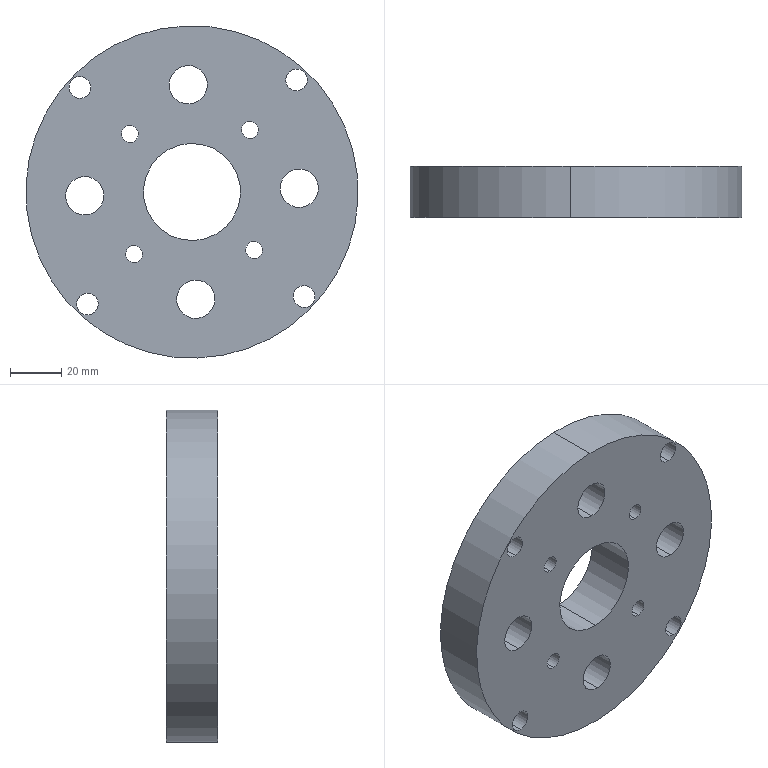Component | SolidWorks | CylindricalUpperFlangePlate-3 | 1 solid | 106 faces | box 130 x 20 x 130 mm | volume 218549 mm3 | cylinder 68 | cone 32 | plane 6 | commonest cylinder face diameters 3 x32 8.5 x8 11 x8 6.6 x8 15 x8 38 x2 130 x2